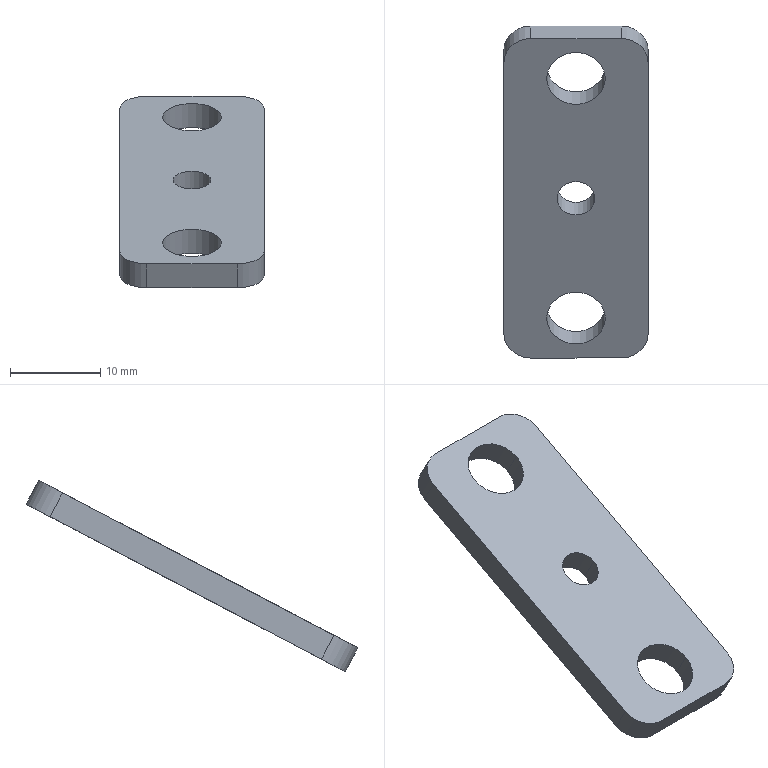Component | SolidWorks | SDACylinderSpringPressurePlate-1 | 1 solid | 16 faces | box 16 x 36.81 x 21.25 mm | volume 1656 mm3 | cylinder 10 | plane 6 | commonest cylinder face diameters 6.5 x4 6 x4 4.2 x2
STEP:
#1=COLOUR_RGB('',0.7922,0.8196,0.9333);
#2=FILL_AREA_STYLE_COLOUR('',#1);
#3=FILL_AREA_STYLE('',(#2));
#4=SURFACE_STYLE_FILL_AREA(#3);
#5=SURFACE_SIDE_STYLE('',(#4));
#6=SURFACE_STYLE_USAGE(.BOTH.,#5);
#7=PRESENTATION_STYLE_ASSIGNMENT((#6));
#8=CARTESIAN_POINT('',(-8.906,-1.43,7.835));
#9=VERTEX_POINT('',#8);
#10=CARTESIAN_POINT('',(-9.072,-1.43,7.835));
#11=VERTEX_POINT('',#10);
#12=CARTESIAN_POINT('',(-8.989,-1.43,7.835));
#13=DIRECTION('',(-0.,0.4648,-0.8854));
#14=DIRECTION('',(-1.,-0.,0.));
#15=AXIS2_PLACEMENT_3D('',#12,#13,#14);
#16=CIRCLE('',#15,0.08268);
#17=EDGE_CURVE('',#9,#11,#16,.T.);
#18=ORIENTED_EDGE('',*,*,#17,.T.);
#19=CARTESIAN_POINT('',(-9.072,-1.484,7.939));
#20=VERTEX_POINT('',#19);
#21=CARTESIAN_POINT('',(-9.072,-1.484,7.939));
#22=DIRECTION('',(0.,-0.4648,0.8854));
#23=VECTOR('',#22,39.37);
#24=LINE('',#21,#23);
#25=EDGE_CURVE('',#11,#20,#24,.T.);
#26=ORIENTED_EDGE('',*,*,#25,.T.);
#27=CARTESIAN_POINT('',(-8.906,-1.484,7.939));
#28=VERTEX_POINT('',#27);
#29=CARTESIAN_POINT('',(-8.989,-1.484,7.939));
#30=DIRECTION('',(0.,-0.4648,0.8854));
#31=DIRECTION('',(1.,0.,0.));
#32=AXIS2_PLACEMENT_3D('',#29,#30,#31);
#33=CIRCLE('',#32,0.08268);
#34=EDGE_CURVE('',#20,#28,#33,.T.);
#35=ORIENTED_EDGE('',*,*,#34,.T.);
#36=CARTESIAN_POINT('',(-8.906,-1.484,7.939));
#37=DIRECTION('',(0.,-0.4648,0.8854));
#38=VECTOR('',#37,39.37);
#39=LINE('',#36,#38);
#40=EDGE_CURVE('',#9,#28,#39,.T.);
#41=ORIENTED_EDGE('',*,*,#40,.F.);
#42=EDGE_LOOP('',(#18,#26,#35,#41));
#43=FACE_OUTER_BOUND('',#42,.T.);
#44=CARTESIAN_POINT('',(-8.989,-1.484,7.939));
#45=DIRECTION('',(0.,-0.4648,0.8854));
#46=DIRECTION('',(1.,0.,0.));
#47=AXIS2_PLACEMENT_3D('',#44,#45,#46);
#48=CYLINDRICAL_SURFACE('',#47,0.08268);
#49=ADVANCED_FACE('',(#43),#48,.F.);
#50=CARTESIAN_POINT('',(-8.861,-0.9067,8.109));
#51=VERTEX_POINT('',#50);
#52=CARTESIAN_POINT('',(-9.117,-0.9067,8.109));
#53=VERTEX_POINT('',#52);
#54=CARTESIAN_POINT('',(-8.989,-0.9067,8.109));
#55=DIRECTION('',(-0.,0.4648,-0.8854));
#56=DIRECTION('',(-1.,-0.,0.));
#57=AXIS2_PLACEMENT_3D('',#54,#55,#56);
#58=CIRCLE('',#57,0.128);
#59=EDGE_CURVE('',#51,#53,#58,.T.);
#60=ORIENTED_EDGE('',*,*,#59,.T.);
#61=CARTESIAN_POINT('',(-9.117,-0.9616,8.214));
#62=VERTEX_POINT('',#61);
#63=CARTESIAN_POINT('',(-9.117,-0.9616,8.214));
#64=DIRECTION('',(0.,-0.4648,0.8854));
#65=VECTOR('',#64,39.37);
#66=LINE('',#63,#65);
#67=EDGE_CURVE('',#53,#62,#66,.T.);
#68=ORIENTED_EDGE('',*,*,#67,.T.);
#69=CARTESIAN_POINT('',(-8.861,-0.9616,8.214));
#70=VERTEX_POINT('',#69);
#71=CARTESIAN_POINT('',(-8.989,-0.9616,8.214));
#72=DIRECTION('',(0.,-0.4648,0.8854));
#73=DIRECTION('',(1.,0.,0.));
#74=AXIS2_PLACEMENT_3D('',#71,#72,#73);
#75=CIRCLE('',#74,0.128);
#76=EDGE_CURVE('',#62,#70,#75,.T.);
#77=ORIENTED_EDGE('',*,*,#76,.T.);
#78=CARTESIAN_POINT('',(-8.861,-0.9616,8.214));
#79=DIRECTION('',(0.,-0.4648,0.8854));
#80=VECTOR('',#79,39.37);
#81=LINE('',#78,#80);
#82=EDGE_CURVE('',#51,#70,#81,.T.);
#83=ORIENTED_EDGE('',*,*,#82,.F.);
#84=EDGE_LOOP('',(#60,#68,#77,#83));
#85=FACE_OUTER_BOUND('',#84,.T.);
#86=CARTESIAN_POINT('',(-8.989,-0.9616,8.214));
#87=DIRECTION('',(0.,-0.4648,0.8854));
#88=DIRECTION('',(1.,0.,0.));
#89=AXIS2_PLACEMENT_3D('',#86,#87,#88);
#90=CYLINDRICAL_SURFACE('',#89,0.128);
#91=ADVANCED_FACE('',(#85),#90,.F.);
#92=CARTESIAN_POINT('',(-8.861,-1.952,7.56));
#93=VERTEX_POINT('',#92);
#94=CARTESIAN_POINT('',(-9.117,-1.952,7.56));
#95=VERTEX_POINT('',#94);
#96=CARTESIAN_POINT('',(-8.989,-1.952,7.56));
#97=DIRECTION('',(-0.,0.4648,-0.8854));
#98=DIRECTION('',(-1.,-0.,0.));
#99=AXIS2_PLACEMENT_3D('',#96,#97,#98);
#100=CIRCLE('',#99,0.128);
#101=EDGE_CURVE('',#93,#95,#100,.T.);
#102=ORIENTED_EDGE('',*,*,#101,.T.);
#103=CARTESIAN_POINT('',(-9.117,-2.007,7.665));
#104=VERTEX_POINT('',#103);
#105=CARTESIAN_POINT('',(-9.117,-2.007,7.665));
#106=DIRECTION('',(0.,-0.4648,0.8854));
#107=VECTOR('',#106,39.37);
#108=LINE('',#105,#107);
#109=EDGE_CURVE('',#95,#104,#108,.T.);
#110=ORIENTED_EDGE('',*,*,#109,.T.);
#111=CARTESIAN_POINT('',(-8.861,-2.007,7.665));
#112=VERTEX_POINT('',#111);
#113=CARTESIAN_POINT('',(-8.989,-2.007,7.665));
#114=DIRECTION('',(0.,-0.4648,0.8854));
#115=DIRECTION('',(1.,0.,0.));
#116=AXIS2_PLACEMENT_3D('',#113,#114,#115);
#117=CIRCLE('',#116,0.128);
#118=EDGE_CURVE('',#104,#112,#117,.T.);
#119=ORIENTED_EDGE('',*,*,#118,.T.);
#120=CARTESIAN_POINT('',(-8.861,-2.007,7.665));
#121=DIRECTION('',(0.,-0.4648,0.8854));
#122=VECTOR('',#121,39.37);
#123=LINE('',#120,#122);
#124=EDGE_CURVE('',#93,#112,#123,.T.);
#125=ORIENTED_EDGE('',*,*,#124,.F.);
#126=EDGE_LOOP('',(#102,#110,#119,#125));
#127=FACE_OUTER_BOUND('',#126,.T.);
#128=CARTESIAN_POINT('',(-8.989,-2.007,7.665));
#129=DIRECTION('',(0.,-0.4648,0.8854));
#130=DIRECTION('',(1.,0.,0.));
#131=AXIS2_PLACEMENT_3D('',#128,#129,#130);
#132=CYLINDRICAL_SURFACE('',#131,0.128);
#133=ADVANCED_FACE('',(#127),#132,.F.);
#134=CARTESIAN_POINT('',(-8.674,-2.022,7.523));
#135=VERTEX_POINT('',#134);
#136=CARTESIAN_POINT('',(-8.674,-0.837,8.146));
#137=VERTEX_POINT('',#136);
#138=CARTESIAN_POINT('',(-8.674,-2.127,7.469));
#139=DIRECTION('',(-0.,0.8854,0.4648));
#140=VECTOR('',#139,39.37);
#141=LINE('',#138,#140);
#142=EDGE_CURVE('',#135,#137,#141,.T.);
#143=ORIENTED_EDGE('',*,*,#142,.T.);
#144=CARTESIAN_POINT('',(-8.674,-0.8919,8.25));
#145=VERTEX_POINT('',#144);
#146=CARTESIAN_POINT('',(-8.674,-0.837,8.146));
#147=DIRECTION('',(0.,-0.4648,0.8854));
#148=VECTOR('',#147,39.37);
#149=LINE('',#146,#148);
#150=EDGE_CURVE('',#137,#145,#149,.T.);
#151=ORIENTED_EDGE('',*,*,#150,.T.);
#152=CARTESIAN_POINT('',(-8.674,-2.077,7.628));
#153=VERTEX_POINT('',#152);
#154=CARTESIAN_POINT('',(-8.674,-2.182,7.573));
#155=DIRECTION('',(-0.,0.8854,0.4648));
#156=VECTOR('',#155,39.37);
#157=LINE('',#154,#156);
#158=EDGE_CURVE('',#153,#145,#157,.T.);
#159=ORIENTED_EDGE('',*,*,#158,.F.);
#160=CARTESIAN_POINT('',(-8.674,-2.022,7.523));
#161=DIRECTION('',(-0.,0.4648,-0.8854));
#162=VECTOR('',#161,39.37);
#163=LINE('',#160,#162);
#164=EDGE_CURVE('',#153,#135,#163,.T.);
#165=ORIENTED_EDGE('',*,*,#164,.T.);
#166=EDGE_LOOP('',(#143,#151,#159,#165));
#167=FACE_OUTER_BOUND('',#166,.T.);
#168=CARTESIAN_POINT('',(-8.674,-2.127,7.469));
#169=DIRECTION('',(1.,0.,-0.));
#170=DIRECTION('',(-0.,0.4648,-0.8854));
#171=AXIS2_PLACEMENT_3D('',#168,#169,#170);
#172=PLANE('',#171);
#173=ADVANCED_FACE('',(#167),#172,.T.);
#174=CARTESIAN_POINT('',(-9.186,-2.127,7.469));
#175=VERTEX_POINT('',#174);
#176=CARTESIAN_POINT('',(-8.792,-2.127,7.469));
#177=VERTEX_POINT('',#176);
#178=CARTESIAN_POINT('',(-9.304,-2.127,7.469));
#179=DIRECTION('',(1.,0.,-0.));
#180=VECTOR('',#179,39.37);
#181=LINE('',#178,#180);
#182=EDGE_CURVE('',#175,#177,#181,.T.);
#183=ORIENTED_EDGE('',*,*,#182,.T.);
#184=CARTESIAN_POINT('',(-8.792,-2.182,7.573));
#185=VERTEX_POINT('',#184);
#186=CARTESIAN_POINT('',(-8.792,-2.127,7.469));
#187=DIRECTION('',(0.,-0.4648,0.8854));
#188=VECTOR('',#187,39.37);
#189=LINE('',#186,#188);
#190=EDGE_CURVE('',#177,#185,#189,.T.);
#191=ORIENTED_EDGE('',*,*,#190,.T.);
#192=CARTESIAN_POINT('',(-9.186,-2.182,7.573));
#193=VERTEX_POINT('',#192);
#194=CARTESIAN_POINT('',(-9.304,-2.182,7.573));
#195=DIRECTION('',(1.,0.,-0.));
#196=VECTOR('',#195,39.37);
#197=LINE('',#194,#196);
#198=EDGE_CURVE('',#193,#185,#197,.T.);
#199=ORIENTED_EDGE('',*,*,#198,.F.);
#200=CARTESIAN_POINT('',(-9.186,-2.127,7.469));
#201=DIRECTION('',(-0.,0.4648,-0.8854));
#202=VECTOR('',#201,39.37);
#203=LINE('',#200,#202);
#204=EDGE_CURVE('',#193,#175,#203,.T.);
#205=ORIENTED_EDGE('',*,*,#204,.T.);
#206=EDGE_LOOP('',(#183,#191,#199,#205));
#207=FACE_OUTER_BOUND('',#206,.T.);
#208=CARTESIAN_POINT('',(-9.304,-2.127,7.469));
#209=DIRECTION('',(0.,-0.8854,-0.4648));
#210=DIRECTION('',(-0.,0.4648,-0.8854));
#211=AXIS2_PLACEMENT_3D('',#208,#209,#210);
#212=PLANE('',#211);
#213=ADVANCED_FACE('',(#207),#212,.T.);
#214=CARTESIAN_POINT('',(-9.304,-0.837,8.146));
#215=VERTEX_POINT('',#214);
#216=CARTESIAN_POINT('',(-9.304,-2.022,7.523));
#217=VERTEX_POINT('',#216);
#218=CARTESIAN_POINT('',(-9.304,-2.127,7.469));
#219=DIRECTION('',(0.,-0.8854,-0.4648));
#220=VECTOR('',#219,39.37);
#221=LINE('',#218,#220);
#222=EDGE_CURVE('',#215,#217,#221,.T.);
#223=ORIENTED_EDGE('',*,*,#222,.T.);
#224=CARTESIAN_POINT('',(-9.304,-2.077,7.628));
#225=VERTEX_POINT('',#224);
#226=CARTESIAN_POINT('',(-9.304,-2.022,7.523));
#227=DIRECTION('',(0.,-0.4648,0.8854));
#228=VECTOR('',#227,39.37);
#229=LINE('',#226,#228);
#230=EDGE_CURVE('',#217,#225,#229,.T.);
#231=ORIENTED_EDGE('',*,*,#230,.T.);
#232=CARTESIAN_POINT('',(-9.304,-0.8919,8.25));
#233=VERTEX_POINT('',#232);
#234=CARTESIAN_POINT('',(-9.304,-2.182,7.573));
#235=DIRECTION('',(0.,-0.8854,-0.4648));
#236=VECTOR('',#235,39.37);
#237=LINE('',#234,#236);
#238=EDGE_CURVE('',#233,#225,#237,.T.);
#239=ORIENTED_EDGE('',*,*,#238,.F.);
#240=CARTESIAN_POINT('',(-9.304,-0.837,8.146));
#241=DIRECTION('',(-0.,0.4648,-0.8854));
#242=VECTOR('',#241,39.37);
#243=LINE('',#240,#242);
#244=EDGE_CURVE('',#233,#215,#243,.T.);
#245=ORIENTED_EDGE('',*,*,#244,.T.);
#246=EDGE_LOOP('',(#223,#231,#239,#245));
#247=FACE_OUTER_BOUND('',#246,.T.);
#248=CARTESIAN_POINT('',(-9.304,-2.127,7.469));
#249=DIRECTION('',(-1.,-0.,0.));
#250=DIRECTION('',(0.,-0.4648,0.8854));
#251=AXIS2_PLACEMENT_3D('',#248,#249,#250);
#252=PLANE('',#251);
#253=ADVANCED_FACE('',(#247),#252,.T.);
#254=CARTESIAN_POINT('',(-8.792,-0.7873,8.305));
#255=VERTEX_POINT('',#254);
#256=CARTESIAN_POINT('',(-9.186,-0.7873,8.305));
#257=VERTEX_POINT('',#256);
#258=CARTESIAN_POINT('',(-9.304,-0.7873,8.305));
#259=DIRECTION('',(-1.,-0.,0.));
#260=VECTOR('',#259,39.37);
#261=LINE('',#258,#260);
#262=EDGE_CURVE('',#255,#257,#261,.T.);
#263=ORIENTED_EDGE('',*,*,#262,.F.);
#264=CARTESIAN_POINT('',(-8.792,-0.7324,8.201));
#265=VERTEX_POINT('',#264);
#266=CARTESIAN_POINT('',(-8.792,-0.7324,8.201));
#267=DIRECTION('',(-0.,0.4648,-0.8854));
#268=VECTOR('',#267,39.37);
#269=LINE('',#266,#268);
#270=EDGE_CURVE('',#255,#265,#269,.T.);
#271=ORIENTED_EDGE('',*,*,#270,.T.);
#272=CARTESIAN_POINT('',(-9.186,-0.7324,8.201));
#273=VERTEX_POINT('',#272);
#274=CARTESIAN_POINT('',(-9.304,-0.7324,8.201));
#275=DIRECTION('',(-1.,-0.,0.));
#276=VECTOR('',#275,39.37);
#277=LINE('',#274,#276);
#278=EDGE_CURVE('',#265,#273,#277,.T.);
#279=ORIENTED_EDGE('',*,*,#278,.T.);
#280=CARTESIAN_POINT('',(-9.186,-0.7324,8.201));
#281=DIRECTION('',(0.,-0.4648,0.8854));
#282=VECTOR('',#281,39.37);
#283=LINE('',#280,#282);
#284=EDGE_CURVE('',#273,#257,#283,.T.);
#285=ORIENTED_EDGE('',*,*,#284,.T.);
#286=EDGE_LOOP('',(#263,#271,#279,#285));
#287=FACE_OUTER_BOUND('',#286,.T.);
#288=CARTESIAN_POINT('',(-9.304,-0.7324,8.201));
#289=DIRECTION('',(-0.,0.8854,0.4648));
#290=DIRECTION('',(0.,-0.4648,0.8854));
#291=AXIS2_PLACEMENT_3D('',#288,#289,#290);
#292=PLANE('',#291);
#293=ADVANCED_FACE('',(#287),#292,.T.);
#294=ORIENTED_EDGE('',*,*,#17,.F.);
#295=CARTESIAN_POINT('',(-8.989,-1.43,7.835));
#296=DIRECTION('',(-0.,0.4648,-0.8854));
#297=DIRECTION('',(-1.,-0.,0.));
#298=AXIS2_PLACEMENT_3D('',#295,#296,#297);
#299=CIRCLE('',#298,0.08268);
#300=EDGE_CURVE('',#11,#9,#299,.T.);
#301=ORIENTED_EDGE('',*,*,#300,.F.);
#302=EDGE_LOOP('',(#294,#301));
#303=FACE_BOUND('',#302,.T.);
#304=ORIENTED_EDGE('',*,*,#59,.F.);
#305=CARTESIAN_POINT('',(-8.989,-0.9067,8.109));
#306=DIRECTION('',(-0.,0.4648,-0.8854));
#307=DIRECTION('',(-1.,-0.,0.));
#308=AXIS2_PLACEMENT_3D('',#305,#306,#307);
#309=CIRCLE('',#308,0.128);
#310=EDGE_CURVE('',#53,#51,#309,.T.);
#311=ORIENTED_EDGE('',*,*,#310,.F.);
#312=EDGE_LOOP('',(#304,#311));
#313=FACE_BOUND('',#312,.T.);
#314=ORIENTED_EDGE('',*,*,#101,.F.);
#315=CARTESIAN_POINT('',(-8.989,-1.952,7.56));
#316=DIRECTION('',(-0.,0.4648,-0.8854));
#317=DIRECTION('',(-1.,-0.,0.));
#318=AXIS2_PLACEMENT_3D('',#315,#316,#317);
#319=CIRCLE('',#318,0.128);
#320=EDGE_CURVE('',#95,#93,#319,.T.);
#321=ORIENTED_EDGE('',*,*,#320,.F.);
#322=EDGE_LOOP('',(#314,#321));
#323=FACE_BOUND('',#322,.T.);
#324=ORIENTED_EDGE('',*,*,#278,.F.);
#325=CARTESIAN_POINT('',(-8.792,-0.837,8.146));
#326=DIRECTION('',(-0.,0.4648,-0.8854));
#327=DIRECTION('',(-1.,-0.,0.));
#328=AXIS2_PLACEMENT_3D('',#325,#326,#327);
#329=CIRCLE('',#328,0.1181);
#330=EDGE_CURVE('',#265,#137,#329,.T.);
#331=ORIENTED_EDGE('',*,*,#330,.T.);
#332=ORIENTED_EDGE('',*,*,#142,.F.);
#333=CARTESIAN_POINT('',(-8.792,-2.022,7.523));
#334=DIRECTION('',(-0.,0.4648,-0.8854));
#335=DIRECTION('',(-1.,-0.,0.));
#336=AXIS2_PLACEMENT_3D('',#333,#334,#335);
#337=CIRCLE('',#336,0.1181);
#338=EDGE_CURVE('',#135,#177,#337,.T.);
#339=ORIENTED_EDGE('',*,*,#338,.T.);
#340=ORIENTED_EDGE('',*,*,#182,.F.);
#341=CARTESIAN_POINT('',(-9.186,-2.022,7.523));
#342=DIRECTION('',(-0.,0.4648,-0.8854));
#343=DIRECTION('',(-1.,-0.,0.));
#344=AXIS2_PLACEMENT_3D('',#341,#342,#343);
#345=CIRCLE('',#344,0.1181);
#346=EDGE_CURVE('',#175,#217,#345,.T.);
#347=ORIENTED_EDGE('',*,*,#346,.T.);
#348=ORIENTED_EDGE('',*,*,#222,.F.);
#349=CARTESIAN_POINT('',(-9.186,-0.837,8.146));
#350=DIRECTION('',(-0.,0.4648,-0.8854));
#351=DIRECTION('',(-1.,-0.,0.));
#352=AXIS2_PLACEMENT_3D('',#349,#350,#351);
#353=CIRCLE('',#352,0.1181);
#354=EDGE_CURVE('',#215,#273,#353,.T.);
#355=ORIENTED_EDGE('',*,*,#354,.T.);
#356=EDGE_LOOP('',(#324,#331,#332,#339,#340,#347,#348,#355));
#357=FACE_OUTER_BOUND('',#356,.T.);
#358=CARTESIAN_POINT('',(-8.989,-1.43,7.835));
#359=DIRECTION('',(-0.,0.4648,-0.8854));
#360=DIRECTION('',(-1.,-0.,0.));
#361=AXIS2_PLACEMENT_3D('',#358,#359,#360);
#362=PLANE('',#361);
#363=ADVANCED_FACE('',(#303,#313,#323,#357),#362,.T.);
#364=CARTESIAN_POINT('',(-8.989,-1.484,7.939));
#365=DIRECTION('',(0.,-0.4648,0.8854));
#366=DIRECTION('',(1.,0.,0.));
#367=AXIS2_PLACEMENT_3D('',#364,#365,#366);
#368=CIRCLE('',#367,0.08268);
#369=EDGE_CURVE('',#28,#20,#368,.T.);
#370=ORIENTED_EDGE('',*,*,#369,.F.);
#371=ORIENTED_EDGE('',*,*,#34,.F.);
#372=EDGE_LOOP('',(#370,#371));
#373=FACE_BOUND('',#372,.T.);
#374=CARTESIAN_POINT('',(-8.989,-0.9616,8.214));
#375=DIRECTION('',(0.,-0.4648,0.8854));
#376=DIRECTION('',(1.,0.,0.));
#377=AXIS2_PLACEMENT_3D('',#374,#375,#376);
#378=CIRCLE('',#377,0.128);
#379=EDGE_CURVE('',#70,#62,#378,.T.);
#380=ORIENTED_EDGE('',*,*,#379,.F.);
#381=ORIENTED_EDGE('',*,*,#76,.F.);
#382=EDGE_LOOP('',(#380,#381));
#383=FACE_BOUND('',#382,.T.);
#384=CARTESIAN_POINT('',(-8.989,-2.007,7.665));
#385=DIRECTION('',(0.,-0.4648,0.8854));
#386=DIRECTION('',(1.,0.,0.));
#387=AXIS2_PLACEMENT_3D('',#384,#385,#386);
#388=CIRCLE('',#387,0.128);
#389=EDGE_CURVE('',#112,#104,#388,.T.);
#390=ORIENTED_EDGE('',*,*,#389,.F.);
#391=ORIENTED_EDGE('',*,*,#118,.F.);
#392=EDGE_LOOP('',(#390,#391));
#393=FACE_BOUND('',#392,.T.);
#394=ORIENTED_EDGE('',*,*,#158,.T.);
#395=CARTESIAN_POINT('',(-8.792,-0.8919,8.25));
#396=DIRECTION('',(0.,-0.4648,0.8854));
#397=DIRECTION('',(-1.,-0.,0.));
#398=AXIS2_PLACEMENT_3D('',#395,#396,#397);
#399=CIRCLE('',#398,0.1181);
#400=EDGE_CURVE('',#145,#255,#399,.T.);
#401=ORIENTED_EDGE('',*,*,#400,.T.);
#402=ORIENTED_EDGE('',*,*,#262,.T.);
#403=CARTESIAN_POINT('',(-9.186,-0.8919,8.25));
#404=DIRECTION('',(0.,-0.4648,0.8854));
#405=DIRECTION('',(-1.,-0.,0.));
#406=AXIS2_PLACEMENT_3D('',#403,#404,#405);
#407=CIRCLE('',#406,0.1181);
#408=EDGE_CURVE('',#257,#233,#407,.T.);
#409=ORIENTED_EDGE('',*,*,#408,.T.);
#410=ORIENTED_EDGE('',*,*,#238,.T.);
#411=CARTESIAN_POINT('',(-9.186,-2.077,7.628));
#412=DIRECTION('',(0.,-0.4648,0.8854));
#413=DIRECTION('',(-1.,-0.,0.));
#414=AXIS2_PLACEMENT_3D('',#411,#412,#413);
#415=CIRCLE('',#414,0.1181);
#416=EDGE_CURVE('',#225,#193,#415,.T.);
#417=ORIENTED_EDGE('',*,*,#416,.T.);
#418=ORIENTED_EDGE('',*,*,#198,.T.);
#419=CARTESIAN_POINT('',(-8.792,-2.077,7.628));
#420=DIRECTION('',(0.,-0.4648,0.8854));
#421=DIRECTION('',(-1.,-0.,0.));
#422=AXIS2_PLACEMENT_3D('',#419,#420,#421);
#423=CIRCLE('',#422,0.1181);
#424=EDGE_CURVE('',#185,#153,#423,.T.);
#425=ORIENTED_EDGE('',*,*,#424,.T.);
#426=EDGE_LOOP('',(#394,#401,#402,#409,#410,#417,#418,#425));
#427=FACE_OUTER_BOUND('',#426,.T.);
#428=CARTESIAN_POINT('',(-8.989,-1.484,7.939));
#429=DIRECTION('',(-0.,0.4648,-0.8854));
#430=DIRECTION('',(-1.,-0.,0.));
#431=AXIS2_PLACEMENT_3D('',#428,#429,#430);
#432=PLANE('',#431);
#433=ADVANCED_FACE('',(#373,#383,#393,#427),#432,.F.);
#434=ORIENTED_EDGE('',*,*,#109,.F.);
#435=ORIENTED_EDGE('',*,*,#320,.T.);
#436=ORIENTED_EDGE('',*,*,#124,.T.);
#437=ORIENTED_EDGE('',*,*,#389,.T.);
#438=EDGE_LOOP('',(#434,#435,#436,#437));
#439=FACE_OUTER_BOUND('',#438,.T.);
#440=CARTESIAN_POINT('',(-8.989,-2.007,7.665));
#441=DIRECTION('',(0.,-0.4648,0.8854));
#442=DIRECTION('',(1.,0.,0.));
#443=AXIS2_PLACEMENT_3D('',#440,#441,#442);
#444=CYLINDRICAL_SURFACE('',#443,0.128);
#445=ADVANCED_FACE('',(#439),#444,.F.);
#446=ORIENTED_EDGE('',*,*,#67,.F.);
#447=ORIENTED_EDGE('',*,*,#310,.T.);
#448=ORIENTED_EDGE('',*,*,#82,.T.);
#449=ORIENTED_EDGE('',*,*,#379,.T.);
#450=EDGE_LOOP('',(#446,#447,#448,#449));
#451=FACE_OUTER_BOUND('',#450,.T.);
#452=CARTESIAN_POINT('',(-8.989,-0.9616,8.214));
#453=DIRECTION('',(0.,-0.4648,0.8854));
#454=DIRECTION('',(1.,0.,0.));
#455=AXIS2_PLACEMENT_3D('',#452,#453,#454);
#456=CYLINDRICAL_SURFACE('',#455,0.128);
#457=ADVANCED_FACE('',(#451),#456,.F.);
#458=ORIENTED_EDGE('',*,*,#330,.F.);
#459=ORIENTED_EDGE('',*,*,#270,.F.);
#460=ORIENTED_EDGE('',*,*,#400,.F.);
#461=ORIENTED_EDGE('',*,*,#150,.F.);
#462=EDGE_LOOP('',(#458,#459,#460,#461));
#463=FACE_OUTER_BOUND('',#462,.T.);
#464=CARTESIAN_POINT('',(-8.792,-0.837,8.146));
#465=DIRECTION('',(0.,-0.4648,0.8854));
#466=DIRECTION('',(1.,0.,0.));
#467=AXIS2_PLACEMENT_3D('',#464,#465,#466);
#468=CYLINDRICAL_SURFACE('',#467,0.1181);
#469=ADVANCED_FACE('',(#463),#468,.T.);
#470=ORIENTED_EDGE('',*,*,#338,.F.);
#471=ORIENTED_EDGE('',*,*,#164,.F.);
#472=ORIENTED_EDGE('',*,*,#424,.F.);
#473=ORIENTED_EDGE('',*,*,#190,.F.);
#474=EDGE_LOOP('',(#470,#471,#472,#473));
#475=FACE_OUTER_BOUND('',#474,.T.);
#476=CARTESIAN_POINT('',(-8.792,-2.022,7.523));
#477=DIRECTION('',(0.,-0.4648,0.8854));
#478=DIRECTION('',(1.,0.,0.));
#479=AXIS2_PLACEMENT_3D('',#476,#477,#478);
#480=CYLINDRICAL_SURFACE('',#479,0.1181);
#481=ADVANCED_FACE('',(#475),#480,.T.);
#482=ORIENTED_EDGE('',*,*,#346,.F.);
#483=ORIENTED_EDGE('',*,*,#204,.F.);
#484=ORIENTED_EDGE('',*,*,#416,.F.);
#485=ORIENTED_EDGE('',*,*,#230,.F.);
#486=EDGE_LOOP('',(#482,#483,#484,#485));
#487=FACE_OUTER_BOUND('',#486,.T.);
#488=CARTESIAN_POINT('',(-9.186,-2.022,7.523));
#489=DIRECTION('',(0.,-0.4648,0.8854));
#490=DIRECTION('',(1.,0.,0.));
#491=AXIS2_PLACEMENT_3D('',#488,#489,#490);
#492=CYLINDRICAL_SURFACE('',#491,0.1181);
#493=ADVANCED_FACE('',(#487),#492,.T.);
#494=ORIENTED_EDGE('',*,*,#354,.F.);
#495=ORIENTED_EDGE('',*,*,#244,.F.);
#496=ORIENTED_EDGE('',*,*,#408,.F.);
#497=ORIENTED_EDGE('',*,*,#284,.F.);
#498=EDGE_LOOP('',(#494,#495,#496,#497));
#499=FACE_OUTER_BOUND('',#498,.T.);
#500=CARTESIAN_POINT('',(-9.186,-0.837,8.146));
#501=DIRECTION('',(0.,-0.4648,0.8854));
#502=DIRECTION('',(1.,0.,0.));
#503=AXIS2_PLACEMENT_3D('',#500,#501,#502);
#504=CYLINDRICAL_SURFACE('',#503,0.1181);
#505=ADVANCED_FACE('',(#499),#504,.T.);
#506=ORIENTED_EDGE('',*,*,#25,.F.);
#507=ORIENTED_EDGE('',*,*,#300,.T.);
#508=ORIENTED_EDGE('',*,*,#40,.T.);
#509=ORIENTED_EDGE('',*,*,#369,.T.);
#510=EDGE_LOOP('',(#506,#507,#508,#509));
#511=FACE_OUTER_BOUND('',#510,.T.);
#512=CARTESIAN_POINT('',(-8.989,-1.484,7.939));
#513=DIRECTION('',(0.,-0.4648,0.8854));
#514=DIRECTION('',(1.,0.,0.));
#515=AXIS2_PLACEMENT_3D('',#512,#513,#514);
#516=CYLINDRICAL_SURFACE('',#515,0.08268);
#517=ADVANCED_FACE('',(#511),#516,.F.);
#518=CLOSED_SHELL('',(#49,#91,#133,#173,#213,#253,#293,#363,#433,#445,#457,#469,#481,#493,#505,#517));
#519=MANIFOLD_SOLID_BREP('',#518);
#520=STYLED_ITEM('',(#7),#519);
#521=(LENGTH_UNIT()NAMED_UNIT(*)SI_UNIT($,.METRE.));
#522=LENGTH_MEASURE_WITH_UNIT(LENGTH_MEASURE(0.0254),#521);
#523=DIMENSIONAL_EXPONENTS(1.,0.,0.,0.,0.,0.,0.);
#524=(CONVERSION_BASED_UNIT('',#522)LENGTH_UNIT()NAMED_UNIT(#523));
#525=UNCERTAINTY_MEASURE_WITH_UNIT(LENGTH_MEASURE(0.00001),#524,'','');
#526=(NAMED_UNIT(*)PLANE_ANGLE_UNIT()SI_UNIT($,.RADIAN.));
#527=(NAMED_UNIT(*)SI_UNIT($,.STERADIAN.)SOLID_ANGLE_UNIT());
#528=(GEOMETRIC_REPRESENTATION_CONTEXT(3)GLOBAL_UNCERTAINTY_ASSIGNED_CONTEXT((#525))GLOBAL_UNIT_ASSIGNED_CONTEXT((#524,#526,#527))REPRESENTATION_CONTEXT('',''));
#529=MECHANICAL_DESIGN_GEOMETRIC_PRESENTATION_REPRESENTATION('',(#520),#528);
#530=CARTESIAN_POINT('',(0.,0.,0.));
#531=DIRECTION('',(0.,0.,1.));
#532=DIRECTION('',(1.,0.,0.));
#533=AXIS2_PLACEMENT_3D('',#530,#531,#532);
#534=(LENGTH_UNIT()NAMED_UNIT(*)SI_UNIT($,.METRE.));
#535=LENGTH_MEASURE_WITH_UNIT(LENGTH_MEASURE(0.0254),#534);
#536=DIMENSIONAL_EXPONENTS(1.,0.,0.,0.,0.,0.,0.);
#537=(CONVERSION_BASED_UNIT('',#535)LENGTH_UNIT()NAMED_UNIT(#536));
#538=UNCERTAINTY_MEASURE_WITH_UNIT(LENGTH_MEASURE(0.00001),#537,'','');
#539=(NAMED_UNIT(*)PLANE_ANGLE_UNIT()SI_UNIT($,.RADIAN.));
#540=(NAMED_UNIT(*)SI_UNIT($,.STERADIAN.)SOLID_ANGLE_UNIT());
#541=(GEOMETRIC_REPRESENTATION_CONTEXT(3)GLOBAL_UNCERTAINTY_ASSIGNED_CONTEXT((#538))GLOBAL_UNIT_ASSIGNED_CONTEXT((#537,#539,#540))REPRESENTATION_CONTEXT('',''));
#542=ADVANCED_BREP_SHAPE_REPRESENTATION('',(#519,#533),#541);
#543=PRESENTATION_LAYER_ASSIGNMENT('','',(#520));